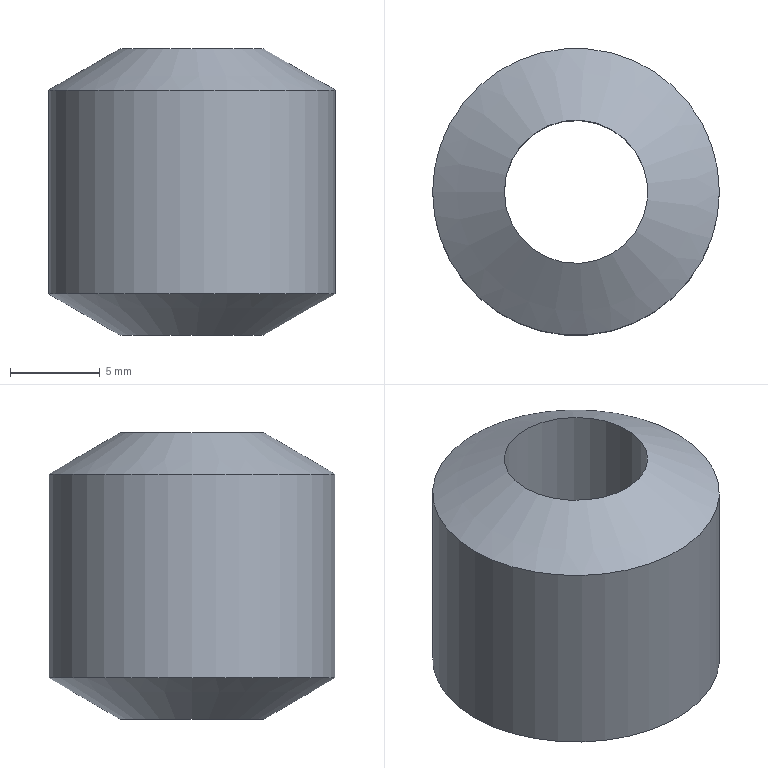Component | NX | PACKING | 1 solid | 4 faces | box 16 x 16 x 16 mm | volume 2026 mm3 | cylinder 2 | cone 2 | commonest cylinder face diameters 16 x1 8 x1
STEP:
#1=CARTESIAN_POINT('',(0.,0.,0.));
#2=DIRECTION('',(0.,0.,1.));
#3=DIRECTION('',(1.,0.,0.));
#4=AXIS2_PLACEMENT_3D('',#1,#2,#3);
#5=CARTESIAN_POINT('',(2.284,5.784,120.309));
#6=VERTEX_POINT('',#5);
#7=CARTESIAN_POINT('',(10.284,5.784,120.309));
#8=DIRECTION('',(0.,0.,1.));
#9=DIRECTION('',(-1.,0.,0.));
#10=AXIS2_PLACEMENT_3D('',#7,#8,#9);
#11=CIRCLE('',#10,8.);
#12=CARTESIAN_POINT('',(10.284,5.784,118.));
#13=DIRECTION('',(0.,0.,1.));
#14=DIRECTION('',(-1.,0.,0.));
#15=AXIS2_PLACEMENT_3D('',#12,#13,#14);
#16=CYLINDRICAL_SURFACE('',#15,8.);
#17=CARTESIAN_POINT('',(0.,2.309));
#18=DIRECTION('',(1.,0.));
#19=VECTOR('',#18,1.);
#20=LINE('',#17,#19);
#21=(GEOMETRIC_REPRESENTATION_CONTEXT(2)PARAMETRIC_REPRESENTATION_CONTEXT()REPRESENTATION_CONTEXT('',''));
#22=DEFINITIONAL_REPRESENTATION('',(#20),#21);
#23=PCURVE('',#16,#22);
#24=CARTESIAN_POINT('',(10.284,5.784,118.));
#25=DIRECTION('',(0.,0.,1.));
#26=DIRECTION('',(-1.,0.,0.));
#27=AXIS2_PLACEMENT_3D('',#24,#25,#26);
#28=CONICAL_SURFACE('',#27,4.,1.047);
#29=CARTESIAN_POINT('',(0.,2.309));
#30=DIRECTION('',(1.,0.));
#31=VECTOR('',#30,1.);
#32=LINE('',#29,#31);
#33=(GEOMETRIC_REPRESENTATION_CONTEXT(2)PARAMETRIC_REPRESENTATION_CONTEXT()REPRESENTATION_CONTEXT('',''));
#34=DEFINITIONAL_REPRESENTATION('',(#32),#33);
#35=PCURVE('',#28,#34);
#36=SURFACE_CURVE('',#11,(#23,#35),.PCURVE_S1.);
#37=EDGE_CURVE('',#6,#6,#36,.T.);
#38=ORIENTED_EDGE('',*,*,#37,.T.);
#39=CARTESIAN_POINT('',(2.284,5.784,131.691));
#40=VERTEX_POINT('',#39);
#41=CARTESIAN_POINT('',(2.284,5.784,120.309));
#42=CARTESIAN_POINT('',(2.284,5.784,131.691));
#43=B_SPLINE_CURVE_WITH_KNOTS('',1,(#41,#42),.UNSPECIFIED.,.F.,.F.,(2,2),(2.309,13.691),.PIECEWISE_BEZIER_KNOTS.);
#44=CARTESIAN_POINT('',(6.283,0.));
#45=DIRECTION('',(0.,1.));
#46=VECTOR('',#45,1.);
#47=LINE('',#44,#46);
#48=(GEOMETRIC_REPRESENTATION_CONTEXT(2)PARAMETRIC_REPRESENTATION_CONTEXT()REPRESENTATION_CONTEXT('',''));
#49=DEFINITIONAL_REPRESENTATION('',(#47),#48);
#50=PCURVE('',#16,#49);
#51=CARTESIAN_POINT('',(0.,0.));
#52=DIRECTION('',(0.,1.));
#53=VECTOR('',#52,1.);
#54=LINE('',#51,#53);
#55=(GEOMETRIC_REPRESENTATION_CONTEXT(2)PARAMETRIC_REPRESENTATION_CONTEXT()REPRESENTATION_CONTEXT('',''));
#56=DEFINITIONAL_REPRESENTATION('',(#54),#55);
#57=PCURVE('',#16,#56);
#58=SEAM_CURVE('',#43,(#50,#57),.PCURVE_S1.);
#59=EDGE_CURVE('',#6,#40,#58,.T.);
#60=ORIENTED_EDGE('',*,*,#59,.T.);
#61=CARTESIAN_POINT('',(10.284,5.784,131.691));
#62=DIRECTION('',(-0.,0.,-1.));
#63=DIRECTION('',(-1.,0.,0.));
#64=AXIS2_PLACEMENT_3D('',#61,#62,#63);
#65=CIRCLE('',#64,8.);
#66=CARTESIAN_POINT('',(6.283,13.691));
#67=DIRECTION('',(-1.,0.));
#68=VECTOR('',#67,1.);
#69=LINE('',#66,#68);
#70=(GEOMETRIC_REPRESENTATION_CONTEXT(2)PARAMETRIC_REPRESENTATION_CONTEXT()REPRESENTATION_CONTEXT('',''));
#71=DEFINITIONAL_REPRESENTATION('',(#69),#70);
#72=PCURVE('',#16,#71);
#73=CARTESIAN_POINT('',(10.284,5.784,134.));
#74=DIRECTION('',(-0.,0.,-1.));
#75=DIRECTION('',(1.,0.,-0.));
#76=AXIS2_PLACEMENT_3D('',#73,#74,#75);
#77=CONICAL_SURFACE('',#76,4.,1.047);
#78=CARTESIAN_POINT('',(3.142,2.309));
#79=DIRECTION('',(1.,0.));
#80=VECTOR('',#79,1.);
#81=LINE('',#78,#80);
#82=(GEOMETRIC_REPRESENTATION_CONTEXT(2)PARAMETRIC_REPRESENTATION_CONTEXT()REPRESENTATION_CONTEXT('',''));
#83=DEFINITIONAL_REPRESENTATION('',(#81),#82);
#84=PCURVE('',#77,#83);
#85=SURFACE_CURVE('',#65,(#72,#84),.PCURVE_S1.);
#86=EDGE_CURVE('',#40,#40,#85,.T.);
#87=ORIENTED_EDGE('',*,*,#86,.T.);
#88=ORIENTED_EDGE('',*,*,#59,.F.);
#89=EDGE_LOOP('',(#38,#60,#87,#88));
#90=FACE_BOUND('',#89,.T.);
#91=ADVANCED_FACE('',(#90),#16,.T.);
#92=CARTESIAN_POINT('',(6.284,5.784,118.));
#93=VERTEX_POINT('',#92);
#94=CARTESIAN_POINT('',(10.284,5.784,118.));
#95=DIRECTION('',(-0.,0.,-1.));
#96=DIRECTION('',(-1.,0.,0.));
#97=AXIS2_PLACEMENT_3D('',#94,#95,#96);
#98=CIRCLE('',#97,4.);
#99=CARTESIAN_POINT('',(10.284,5.784,118.));
#100=DIRECTION('',(0.,0.,1.));
#101=DIRECTION('',(-1.,0.,0.));
#102=AXIS2_PLACEMENT_3D('',#99,#100,#101);
#103=CYLINDRICAL_SURFACE('',#102,4.);
#104=CARTESIAN_POINT('',(6.283,0.));
#105=DIRECTION('',(-1.,0.));
#106=VECTOR('',#105,1.);
#107=LINE('',#104,#106);
#108=(GEOMETRIC_REPRESENTATION_CONTEXT(2)PARAMETRIC_REPRESENTATION_CONTEXT()REPRESENTATION_CONTEXT('',''));
#109=DEFINITIONAL_REPRESENTATION('',(#107),#108);
#110=PCURVE('',#103,#109);
#111=CARTESIAN_POINT('',(6.283,0.));
#112=DIRECTION('',(-1.,0.));
#113=VECTOR('',#112,1.);
#114=LINE('',#111,#113);
#115=(GEOMETRIC_REPRESENTATION_CONTEXT(2)PARAMETRIC_REPRESENTATION_CONTEXT()REPRESENTATION_CONTEXT('',''));
#116=DEFINITIONAL_REPRESENTATION('',(#114),#115);
#117=PCURVE('',#28,#116);
#118=SURFACE_CURVE('',#98,(#110,#117),.PCURVE_S1.);
#119=EDGE_CURVE('',#93,#93,#118,.T.);
#120=ORIENTED_EDGE('',*,*,#119,.F.);
#121=CARTESIAN_POINT('',(6.284,5.784,134.));
#122=VERTEX_POINT('',#121);
#123=CARTESIAN_POINT('',(6.284,5.784,118.));
#124=CARTESIAN_POINT('',(6.284,5.784,134.));
#125=B_SPLINE_CURVE_WITH_KNOTS('',1,(#123,#124),.UNSPECIFIED.,.F.,.F.,(2,2),(0.,16.),.PIECEWISE_BEZIER_KNOTS.);
#126=CARTESIAN_POINT('',(6.283,0.));
#127=DIRECTION('',(0.,1.));
#128=VECTOR('',#127,1.);
#129=LINE('',#126,#128);
#130=(GEOMETRIC_REPRESENTATION_CONTEXT(2)PARAMETRIC_REPRESENTATION_CONTEXT()REPRESENTATION_CONTEXT('',''));
#131=DEFINITIONAL_REPRESENTATION('',(#129),#130);
#132=PCURVE('',#103,#131);
#133=CARTESIAN_POINT('',(0.,0.));
#134=DIRECTION('',(0.,1.));
#135=VECTOR('',#134,1.);
#136=LINE('',#133,#135);
#137=(GEOMETRIC_REPRESENTATION_CONTEXT(2)PARAMETRIC_REPRESENTATION_CONTEXT()REPRESENTATION_CONTEXT('',''));
#138=DEFINITIONAL_REPRESENTATION('',(#136),#137);
#139=PCURVE('',#103,#138);
#140=SEAM_CURVE('',#125,(#132,#139),.PCURVE_S1.);
#141=EDGE_CURVE('',#93,#122,#140,.T.);
#142=ORIENTED_EDGE('',*,*,#141,.T.);
#143=CARTESIAN_POINT('',(10.284,5.784,134.));
#144=DIRECTION('',(0.,0.,1.));
#145=DIRECTION('',(-1.,0.,0.));
#146=AXIS2_PLACEMENT_3D('',#143,#144,#145);
#147=CIRCLE('',#146,4.);
#148=CARTESIAN_POINT('',(0.,16.));
#149=DIRECTION('',(1.,0.));
#150=VECTOR('',#149,1.);
#151=LINE('',#148,#150);
#152=(GEOMETRIC_REPRESENTATION_CONTEXT(2)PARAMETRIC_REPRESENTATION_CONTEXT()REPRESENTATION_CONTEXT('',''));
#153=DEFINITIONAL_REPRESENTATION('',(#151),#152);
#154=PCURVE('',#103,#153);
#155=CARTESIAN_POINT('',(9.425,0.));
#156=DIRECTION('',(-1.,0.));
#157=VECTOR('',#156,1.);
#158=LINE('',#155,#157);
#159=(GEOMETRIC_REPRESENTATION_CONTEXT(2)PARAMETRIC_REPRESENTATION_CONTEXT()REPRESENTATION_CONTEXT('',''));
#160=DEFINITIONAL_REPRESENTATION('',(#158),#159);
#161=PCURVE('',#77,#160);
#162=SURFACE_CURVE('',#147,(#154,#161),.PCURVE_S1.);
#163=EDGE_CURVE('',#122,#122,#162,.T.);
#164=ORIENTED_EDGE('',*,*,#163,.F.);
#165=ORIENTED_EDGE('',*,*,#141,.F.);
#166=EDGE_LOOP('',(#120,#142,#164,#165));
#167=FACE_BOUND('',#166,.F.);
#168=ADVANCED_FACE('',(#167),#103,.F.);
#169=ORIENTED_EDGE('',*,*,#37,.F.);
#170=CARTESIAN_POINT('',(6.284,5.784,118.));
#171=CARTESIAN_POINT('',(2.284,5.784,120.309));
#172=B_SPLINE_CURVE_WITH_KNOTS('',1,(#170,#171),.UNSPECIFIED.,.F.,.F.,(2,2),(0.,4.619),.PIECEWISE_BEZIER_KNOTS.);
#173=CARTESIAN_POINT('',(0.,0.));
#174=DIRECTION('',(0.,1.));
#175=VECTOR('',#174,1.);
#176=LINE('',#173,#175);
#177=(GEOMETRIC_REPRESENTATION_CONTEXT(2)PARAMETRIC_REPRESENTATION_CONTEXT()REPRESENTATION_CONTEXT('',''));
#178=DEFINITIONAL_REPRESENTATION('',(#176),#177);
#179=PCURVE('',#28,#178);
#180=CARTESIAN_POINT('',(6.283,0.));
#181=DIRECTION('',(0.,1.));
#182=VECTOR('',#181,1.);
#183=LINE('',#180,#182);
#184=(GEOMETRIC_REPRESENTATION_CONTEXT(2)PARAMETRIC_REPRESENTATION_CONTEXT()REPRESENTATION_CONTEXT('',''));
#185=DEFINITIONAL_REPRESENTATION('',(#183),#184);
#186=PCURVE('',#28,#185);
#187=SEAM_CURVE('',#172,(#179,#186),.PCURVE_S1.);
#188=EDGE_CURVE('',#93,#6,#187,.T.);
#189=ORIENTED_EDGE('',*,*,#188,.F.);
#190=ORIENTED_EDGE('',*,*,#119,.F.);
#191=ORIENTED_EDGE('',*,*,#188,.T.);
#192=EDGE_LOOP('',(#169,#189,#190,#191));
#193=FACE_BOUND('',#192,.T.);
#194=ADVANCED_FACE('',(#193),#28,.T.);
#195=ORIENTED_EDGE('',*,*,#86,.F.);
#196=CARTESIAN_POINT('',(6.284,5.784,134.));
#197=CARTESIAN_POINT('',(2.284,5.784,131.691));
#198=B_SPLINE_CURVE_WITH_KNOTS('',1,(#196,#197),.UNSPECIFIED.,.F.,.F.,(2,2),(0.,4.619),.PIECEWISE_BEZIER_KNOTS.);
#199=CARTESIAN_POINT('',(3.142,0.));
#200=DIRECTION('',(0.,1.));
#201=VECTOR('',#200,1.);
#202=LINE('',#199,#201);
#203=(GEOMETRIC_REPRESENTATION_CONTEXT(2)PARAMETRIC_REPRESENTATION_CONTEXT()REPRESENTATION_CONTEXT('',''));
#204=DEFINITIONAL_REPRESENTATION('',(#202),#203);
#205=PCURVE('',#77,#204);
#206=CARTESIAN_POINT('',(9.425,0.));
#207=DIRECTION('',(0.,1.));
#208=VECTOR('',#207,1.);
#209=LINE('',#206,#208);
#210=(GEOMETRIC_REPRESENTATION_CONTEXT(2)PARAMETRIC_REPRESENTATION_CONTEXT()REPRESENTATION_CONTEXT('',''));
#211=DEFINITIONAL_REPRESENTATION('',(#209),#210);
#212=PCURVE('',#77,#211);
#213=SEAM_CURVE('',#198,(#205,#212),.PCURVE_S1.);
#214=EDGE_CURVE('',#122,#40,#213,.T.);
#215=ORIENTED_EDGE('',*,*,#214,.F.);
#216=ORIENTED_EDGE('',*,*,#163,.F.);
#217=ORIENTED_EDGE('',*,*,#214,.T.);
#218=EDGE_LOOP('',(#195,#215,#216,#217));
#219=FACE_BOUND('',#218,.T.);
#220=ADVANCED_FACE('',(#219),#77,.T.);
#221=CLOSED_SHELL('',(#91,#168,#194,#220));
#222=MANIFOLD_SOLID_BREP('',#221);
#223=(LENGTH_UNIT()NAMED_UNIT(*)SI_UNIT(.MILLI.,.METRE.));
#224=UNCERTAINTY_MEASURE_WITH_UNIT(LENGTH_MEASURE(0.00001),#223,'','');
#225=(NAMED_UNIT(*)PLANE_ANGLE_UNIT()SI_UNIT($,.RADIAN.));
#226=(NAMED_UNIT(*)SI_UNIT($,.STERADIAN.)SOLID_ANGLE_UNIT());
#227=(GEOMETRIC_REPRESENTATION_CONTEXT(3)GLOBAL_UNCERTAINTY_ASSIGNED_CONTEXT((#224))GLOBAL_UNIT_ASSIGNED_CONTEXT((#223,#225,#226))REPRESENTATION_CONTEXT('',''));
#228=ADVANCED_BREP_SHAPE_REPRESENTATION('',(#4,#222),#227);